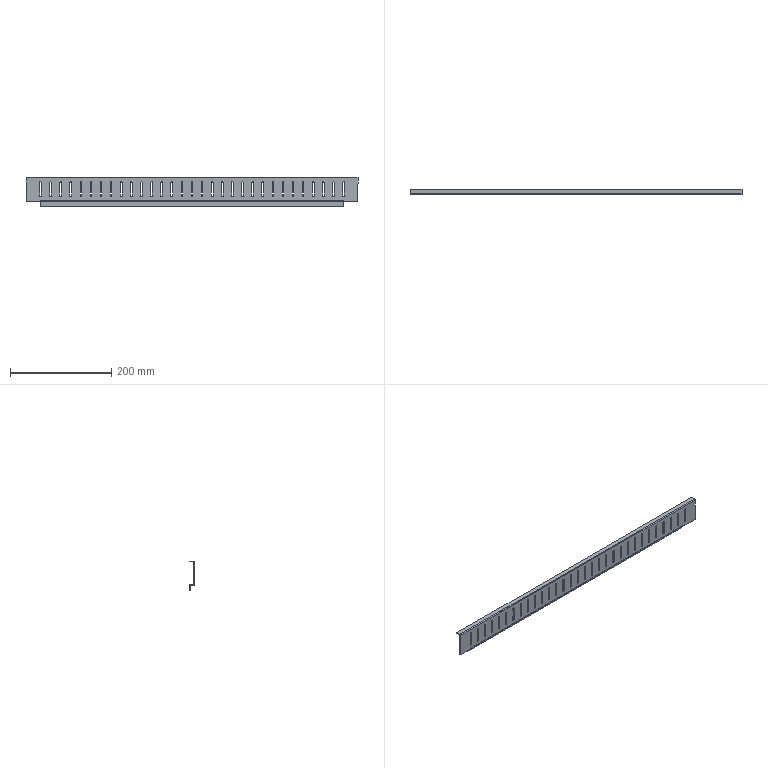Component | SolidWorks | TopCoverFrontSideBeam-1 | 1 solid | 164 faces | volume 67892 mm3 | plane 96 | cylinder 68 | commonest cylinder face diameters 3.2 x65 0.2 x3